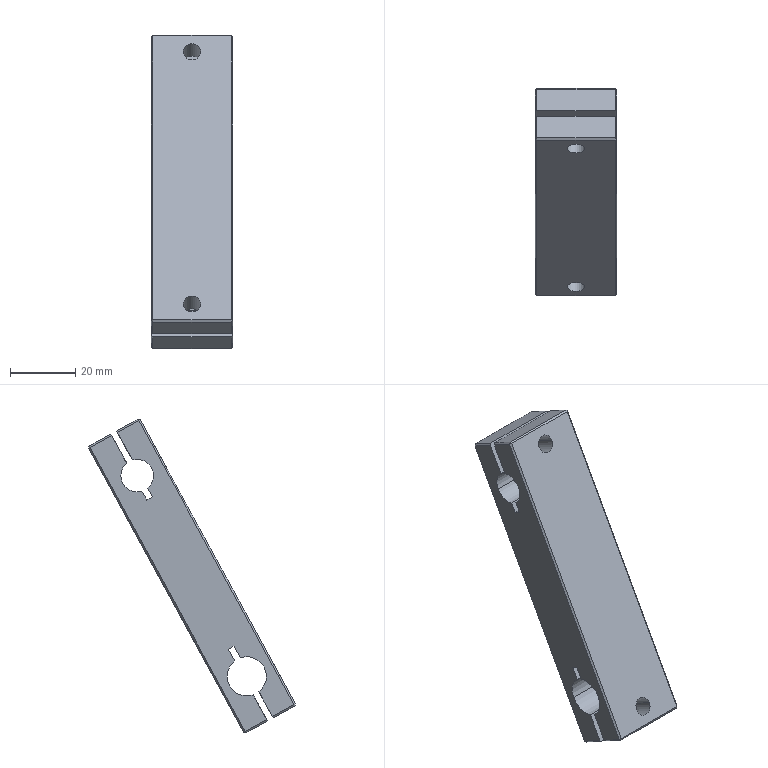Component | SolidWorks | XM-WST05-2010-1 | 1 solid | 56 faces | box 25 x 63.23 x 95.92 mm | volume 38231 mm3 | plane 42 | cylinder 14 | commonest cylinder face diameters 5.5 x4 4.2 x4 12 x3 10 x3
build123d program:
from build123d import *

# Parameters (mm, degrees)
SKETCH1_W                      = 18
SKETCH1_H                      = 100
BOSS_EXTRUDE1_DEPTH            = 25
SKETCH2_R                      = 6
SKETCH2_R_2                    = 5
CUT_EXTRUDE1_DEPTH             = 57.622
SKETCH3_W                      = 2
SKETCH3_H                      = 50
SKETCH3_H_2                    = 46
CUT_EXTRUDE2_DEPTH             = 57.622
M5_TAPPED_HOLE1_D              = 4.2
M5_TAPPED_HOLE1_DEPTH          = 8
F_5_5_5_5_DIAMETER_HOLE1_D     = 5.5
F_5_5_5_5_DIAMETER_HOLE1_DEPTH = 8
CHAMFER2_SIZE                  = 0.5


with BuildPart() as part:
    # Sketch1 → Boss-Extrude1 (new body)
    with BuildSketch(Plane.XY):
        Rectangle(SKETCH1_W, SKETCH1_H)
    extrude(amount=BOSS_EXTRUDE1_DEPTH)

    # Sketch2 → Cut-Extrude1 (cut, through all)
    with BuildSketch(Plane.XY.offset(25)):
        with Locations((0, 35)):
            Circle(SKETCH2_R)
        with Locations((0, -35)):
            Circle(SKETCH2_R_2)
    extrude(amount=-CUT_EXTRUDE1_DEPTH, mode=Mode.SUBTRACT)

    # Sketch3 → Cut-Extrude2 (cut, through all)
    with BuildSketch(Plane.XY.offset(25)):
        with Locations((0, 50)):
            Rectangle(SKETCH3_W, SKETCH3_H)
        with Locations((0, -50)):
            Rectangle(SKETCH3_W, SKETCH3_H_2)
    extrude(amount=-CUT_EXTRUDE2_DEPTH, mode=Mode.SUBTRACT)

    # M5 Tapped Hole1
    with Locations(Plane(origin=(9, 0, 0), x_dir=(0, 0, -1), z_dir=(1, 0, 0))):
        with Locations((-12.5, 44), (-12.5, -44)):
            Hole(M5_TAPPED_HOLE1_D / 2, depth=M5_TAPPED_HOLE1_DEPTH)

    # 5.5 _5.5_ Diameter Hole1
    with Locations(Plane.ZY.offset(9)):
        with Locations((12.5, 44), (12.5, -44)):
            Hole(F_5_5_5_5_DIAMETER_HOLE1_D / 2, depth=F_5_5_5_5_DIAMETER_HOLE1_DEPTH)

    # Chamfer2
    chamfer2_edges = [part.edges().sort_by_distance(p)[0] for p in [
        (9, 0, 25),
        (5, 50, 25),
        (-5, 50, 0),
        (-5, 50, 25),
        (-9, 0, 25),
        (5, 50, 0),
        (9, 0, 0),
        (-5, -50, 0),
        (-9, 0, 0),
        (5, -50, 0),
        (5, -50, 25),
        (-5, -50, 25),
        (-9, 50, 12.5),
        (9, 50, 12.5),
        (9, -50, 12.5),
        (-9, -50, 12.5),
    ]]
    chamfer(chamfer2_edges, length=CHAMFER2_SIZE)


solid = part.part

# Placed as in the assembly
solid = solid.moved(Location((-210.071, 100.939, 390.529), (-118.629, -90, 0)))